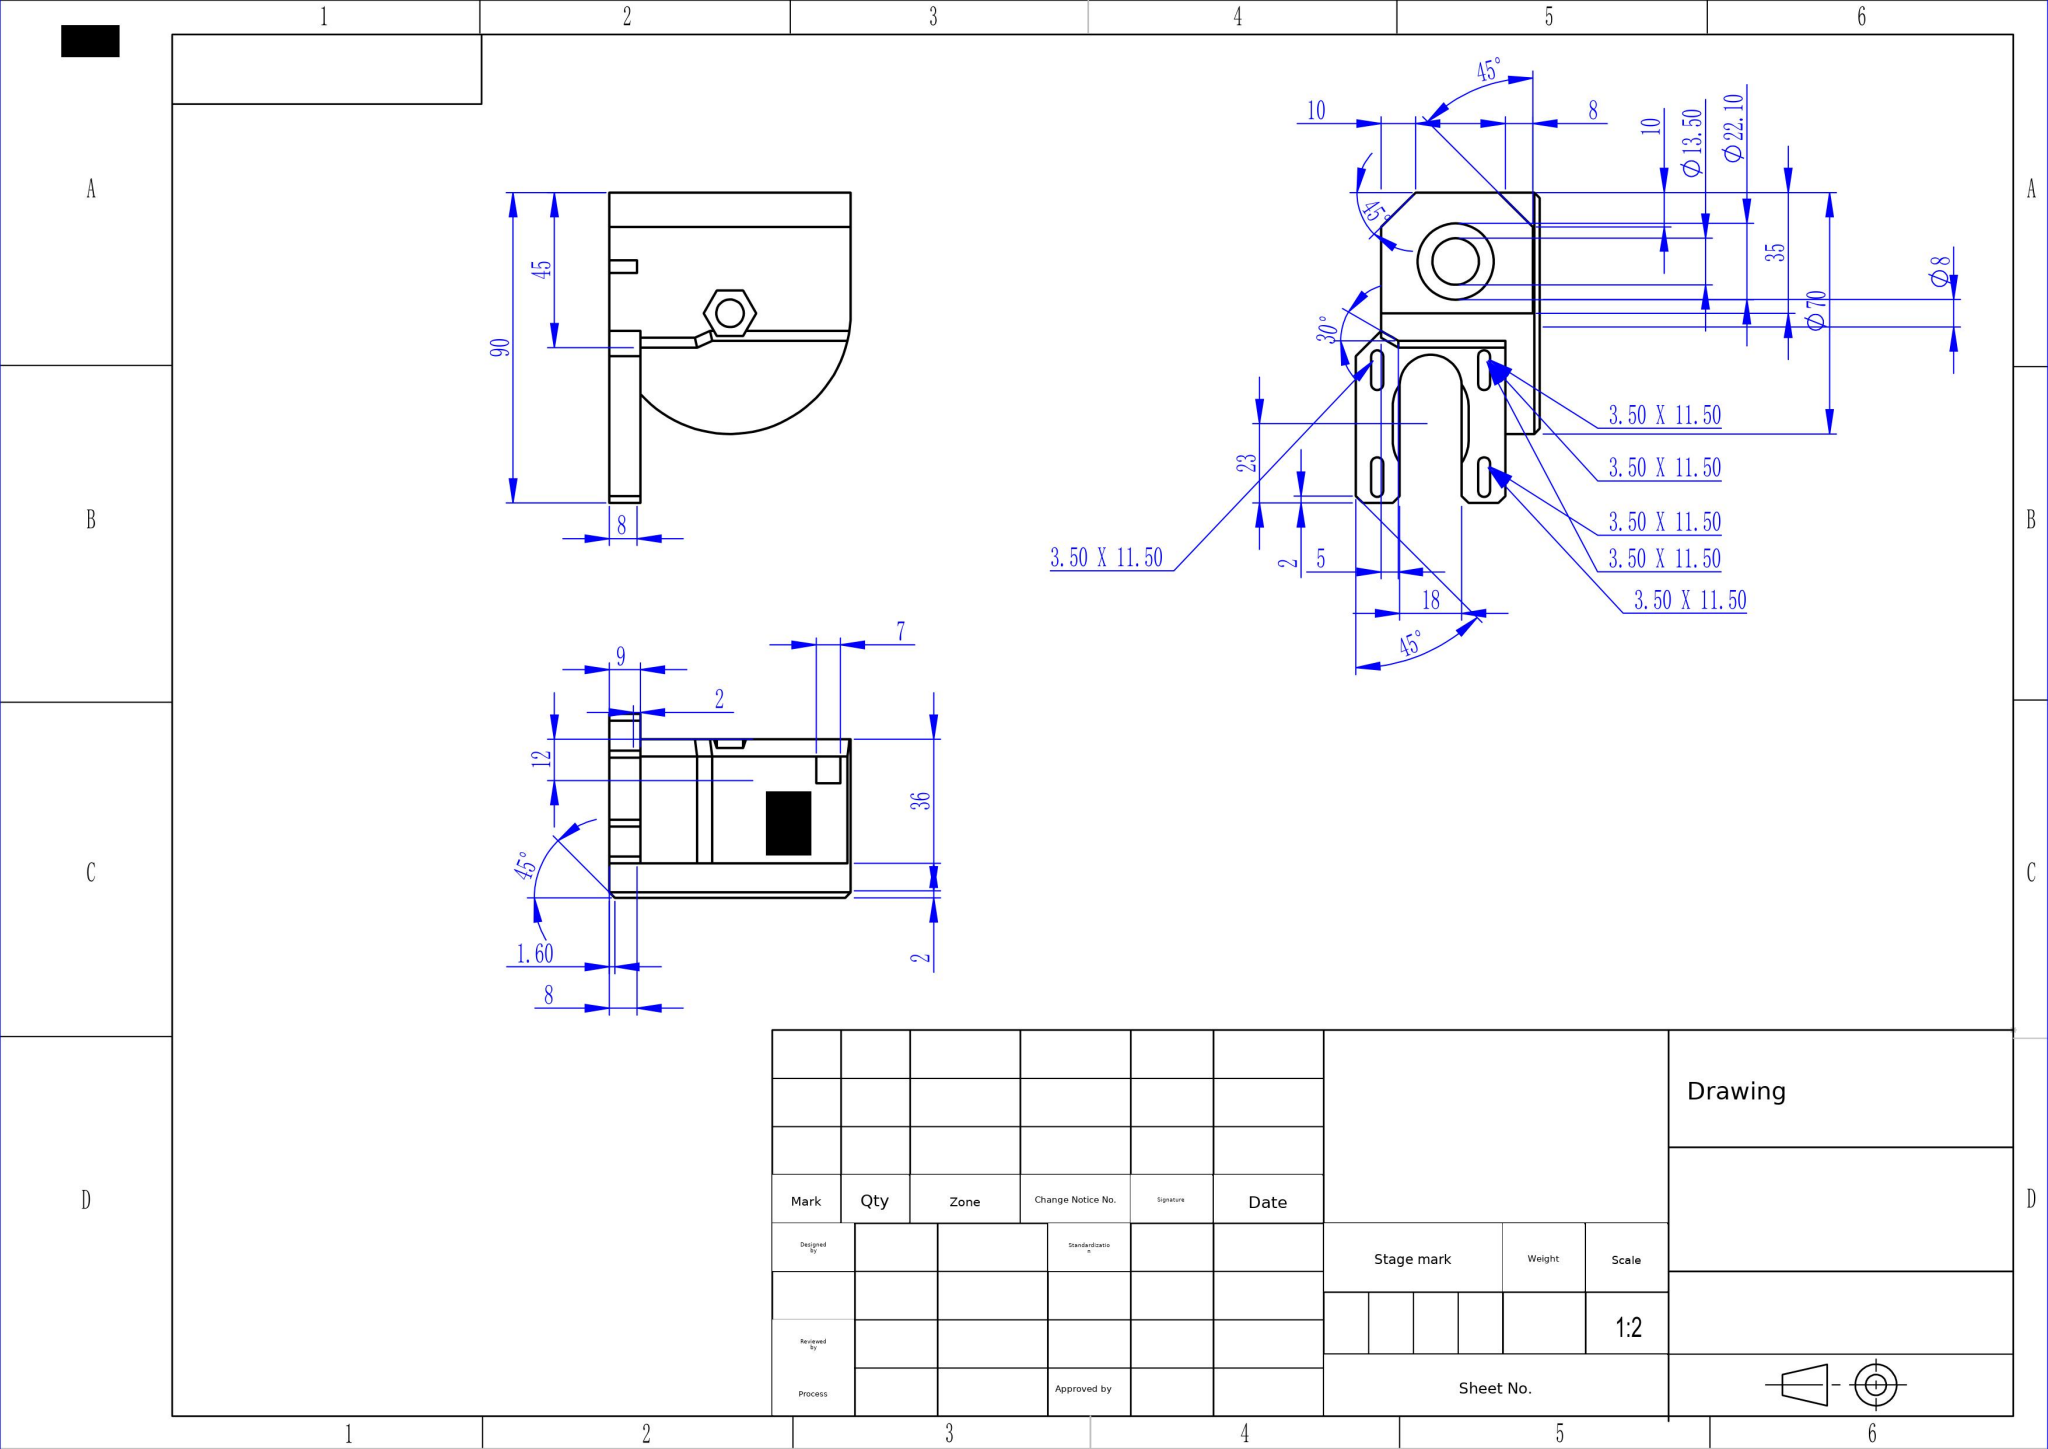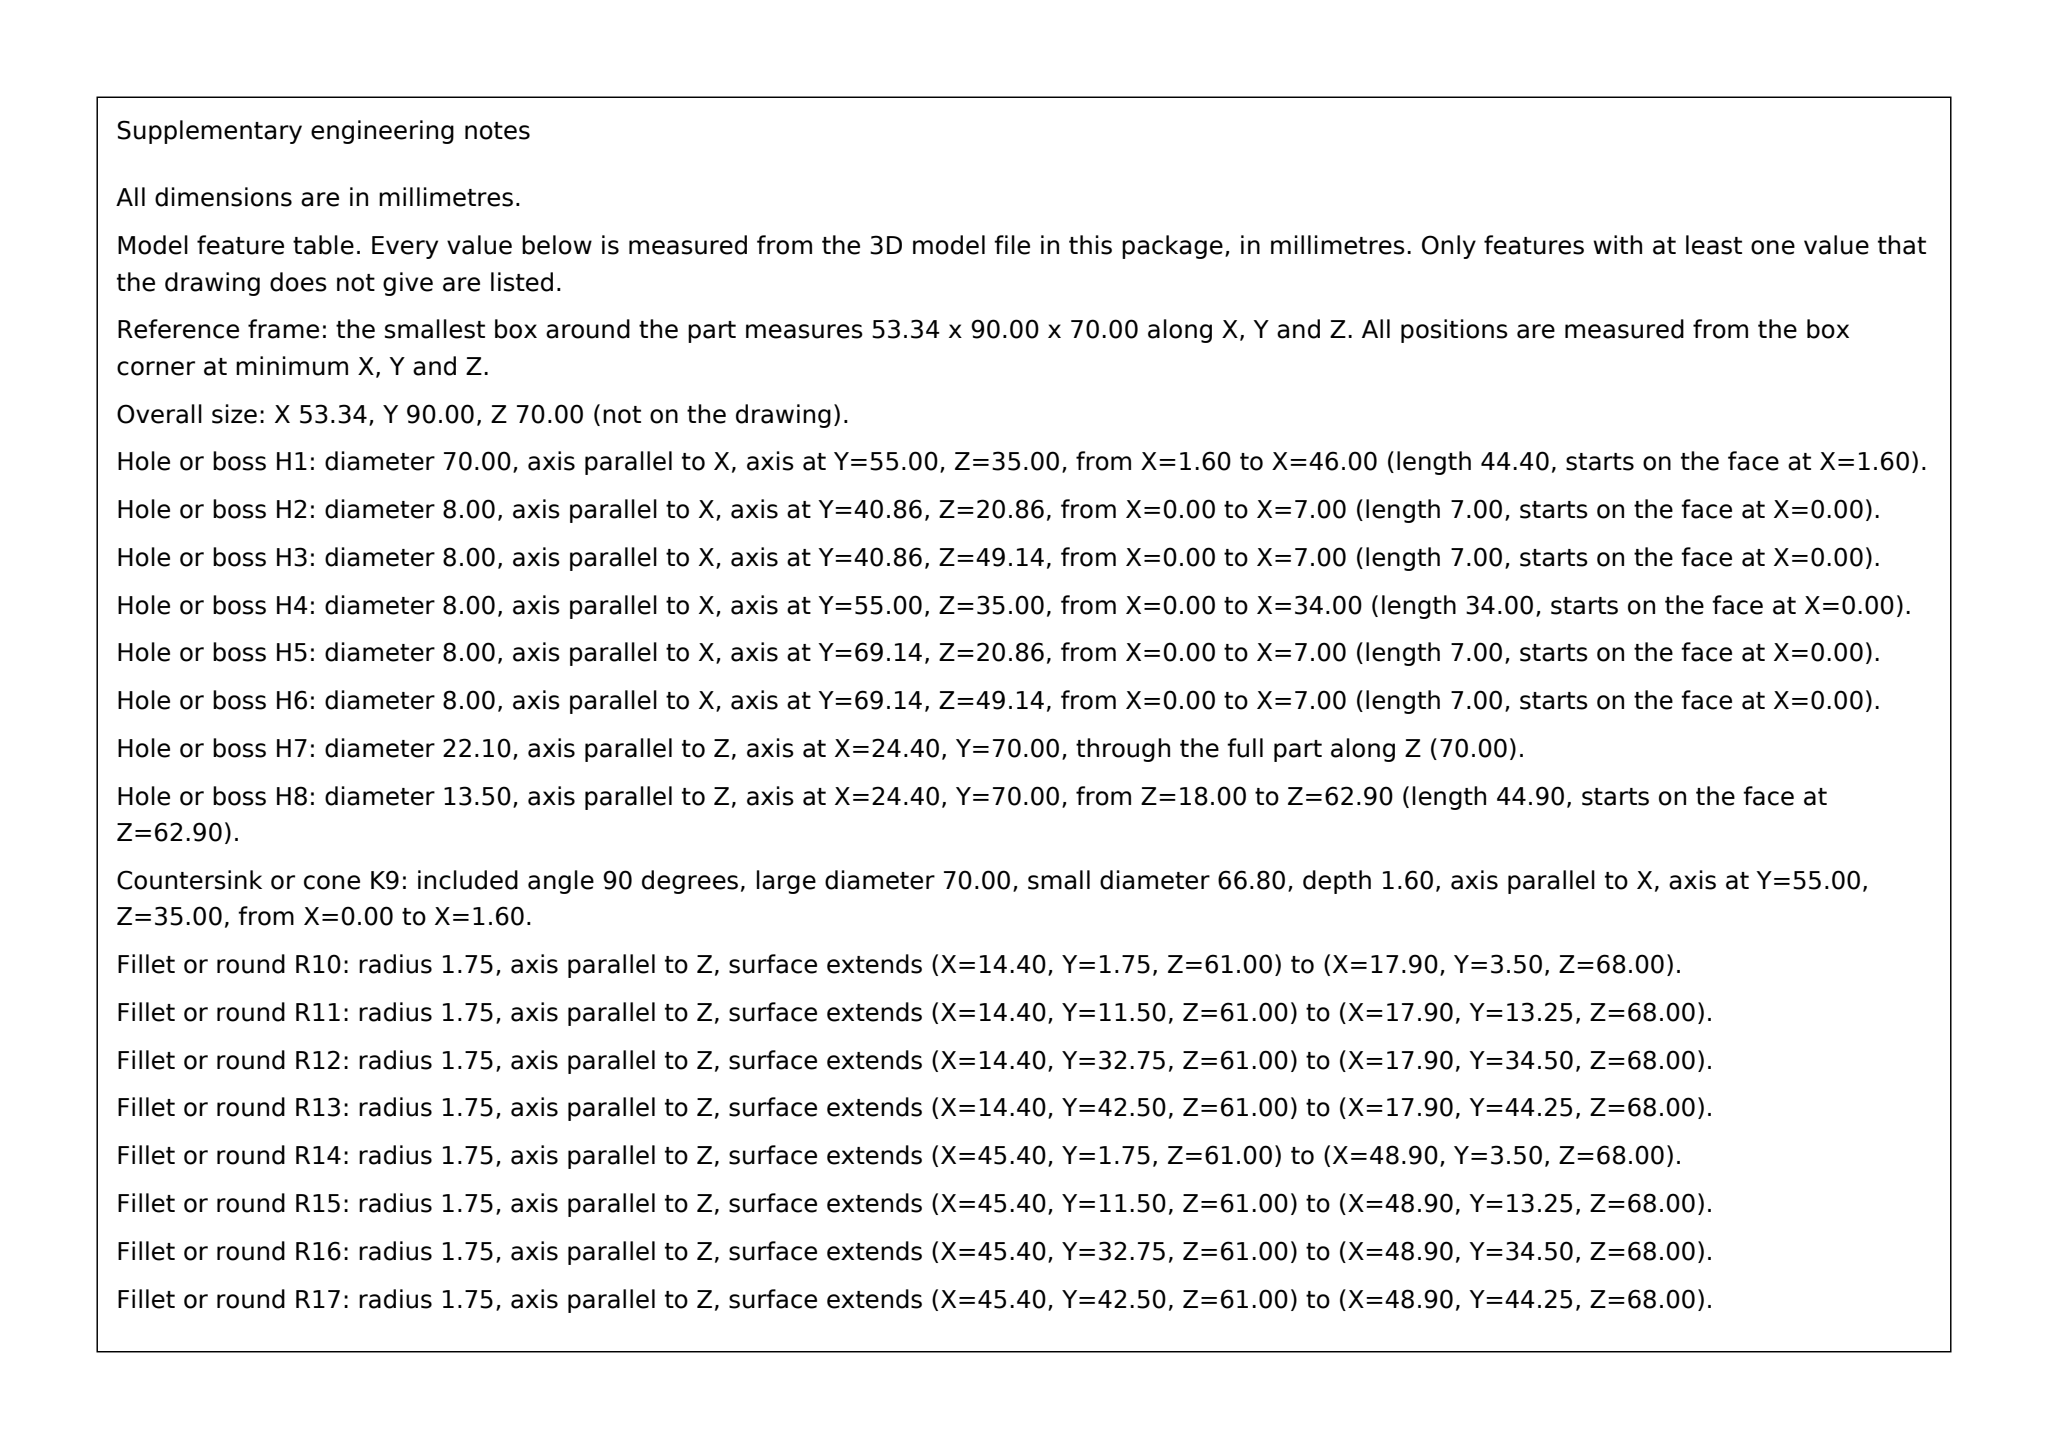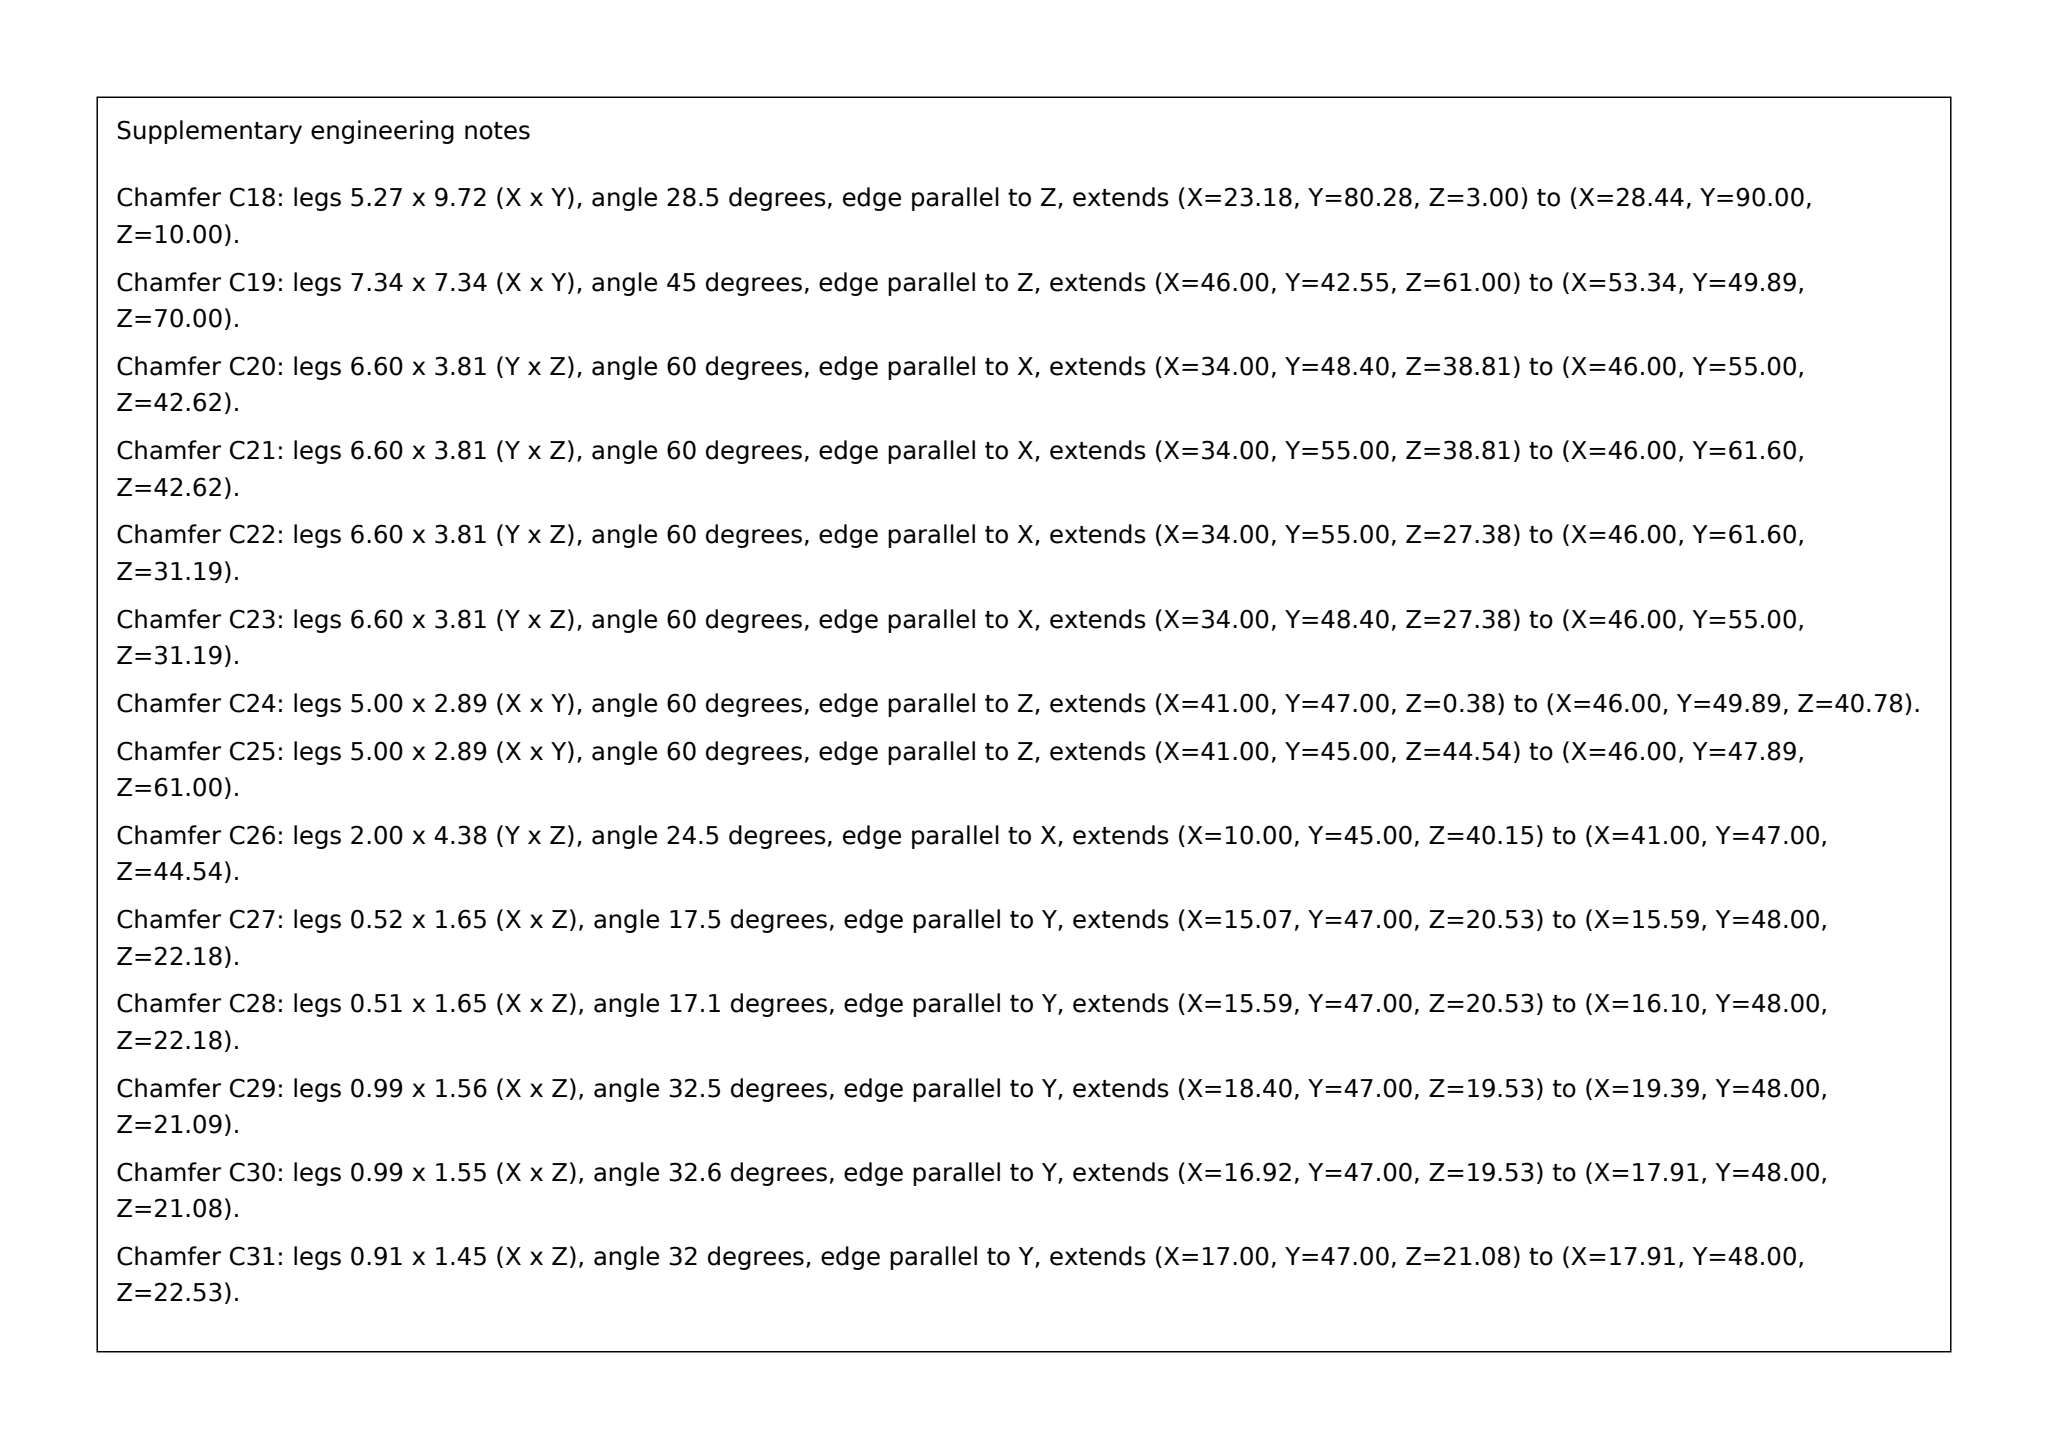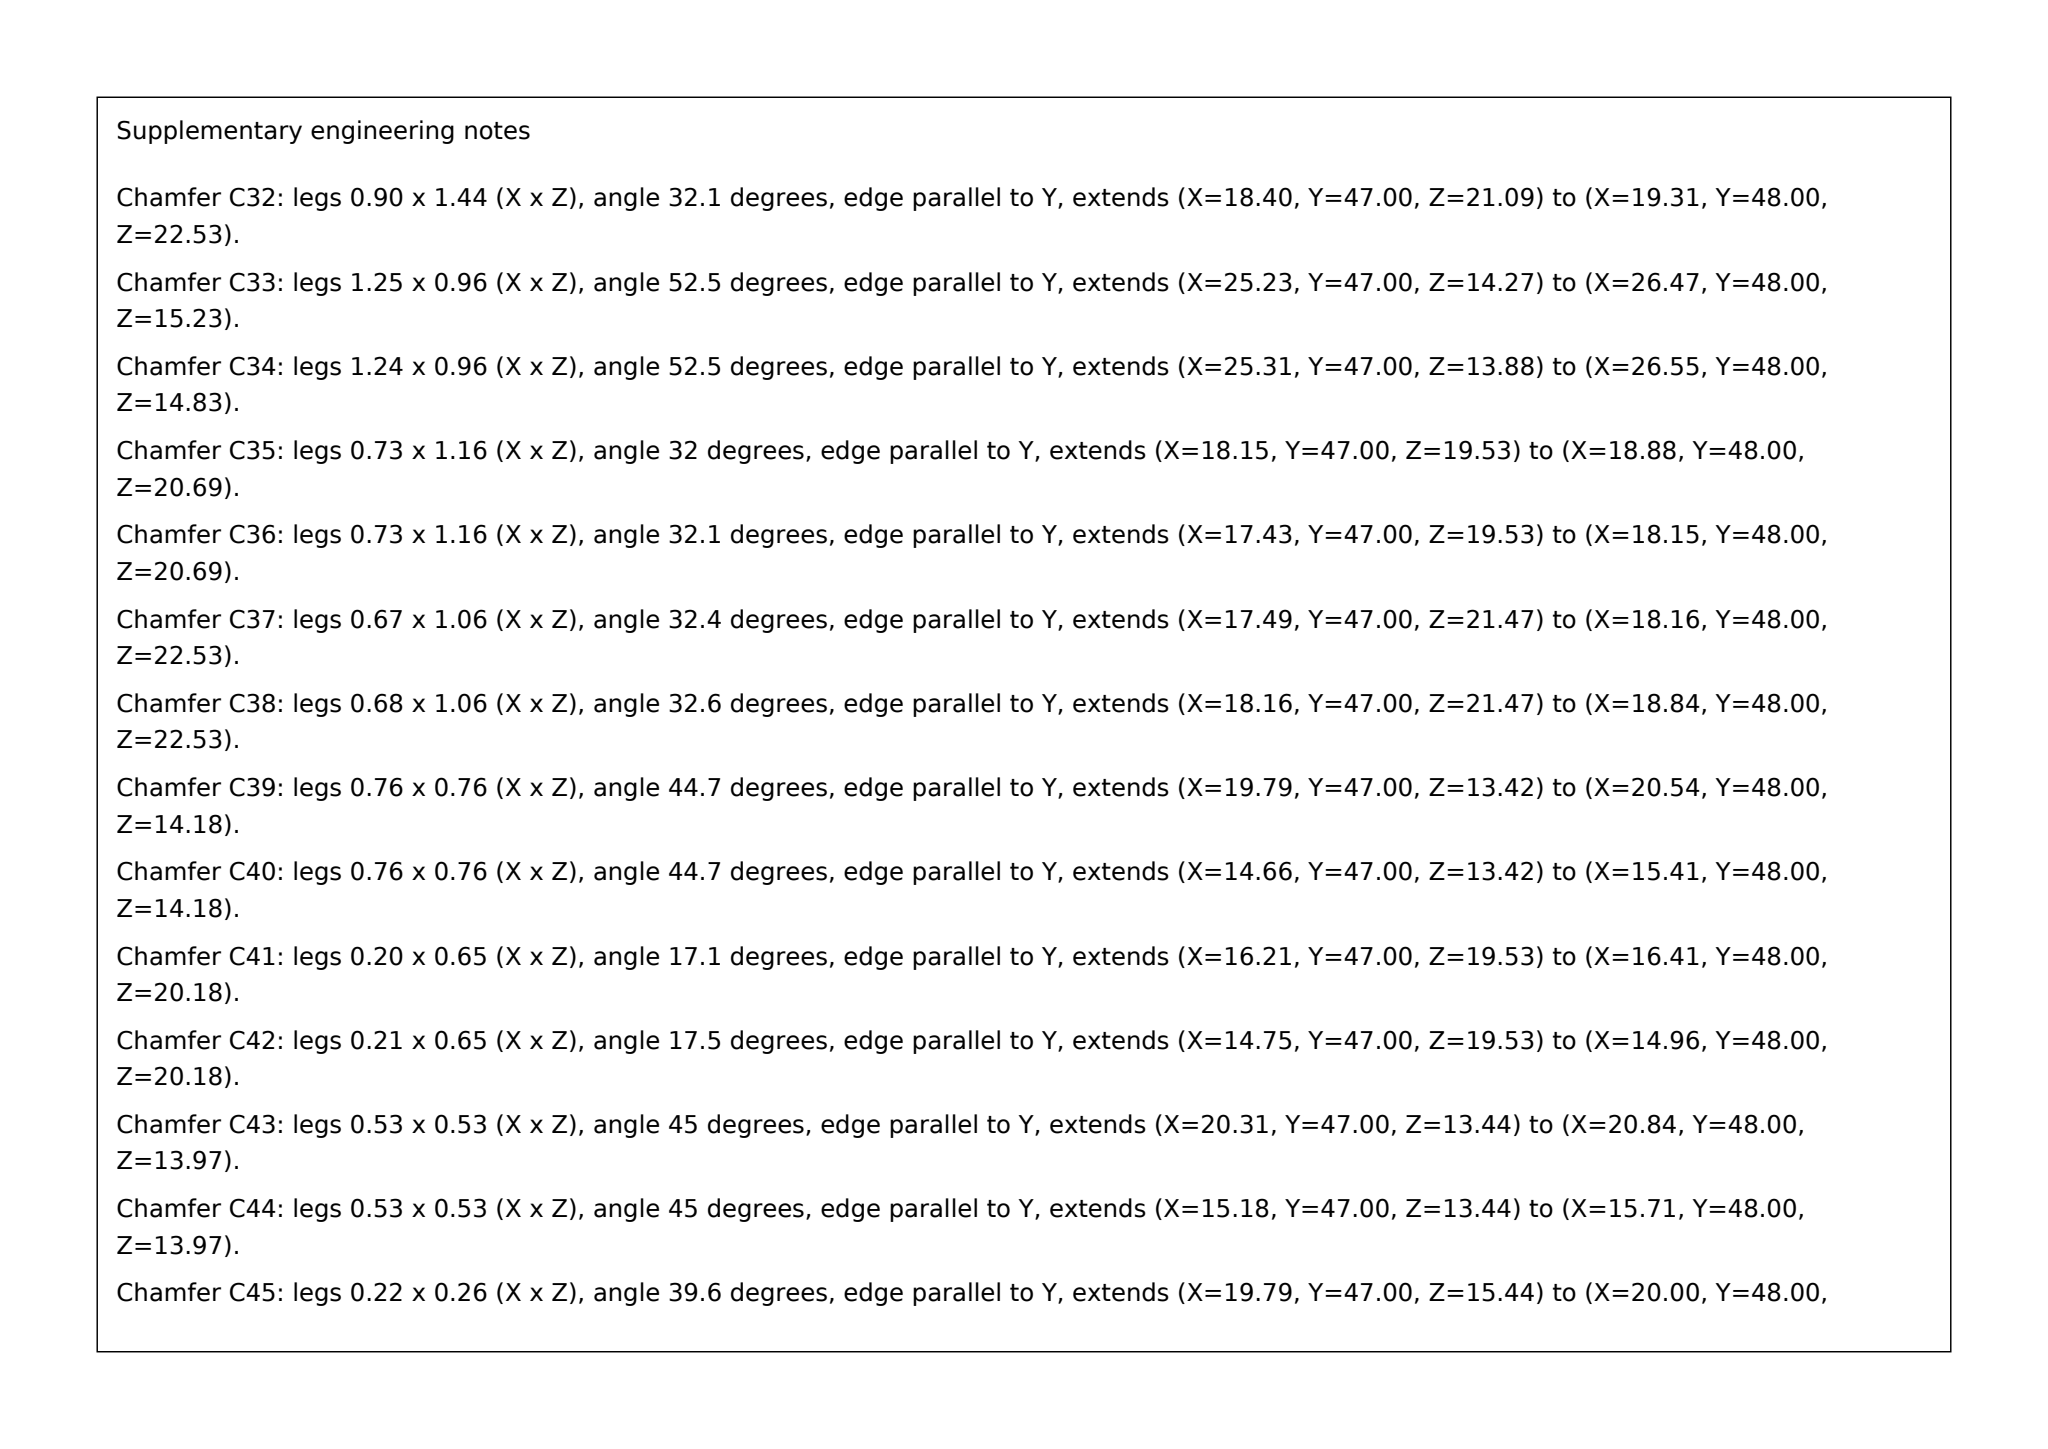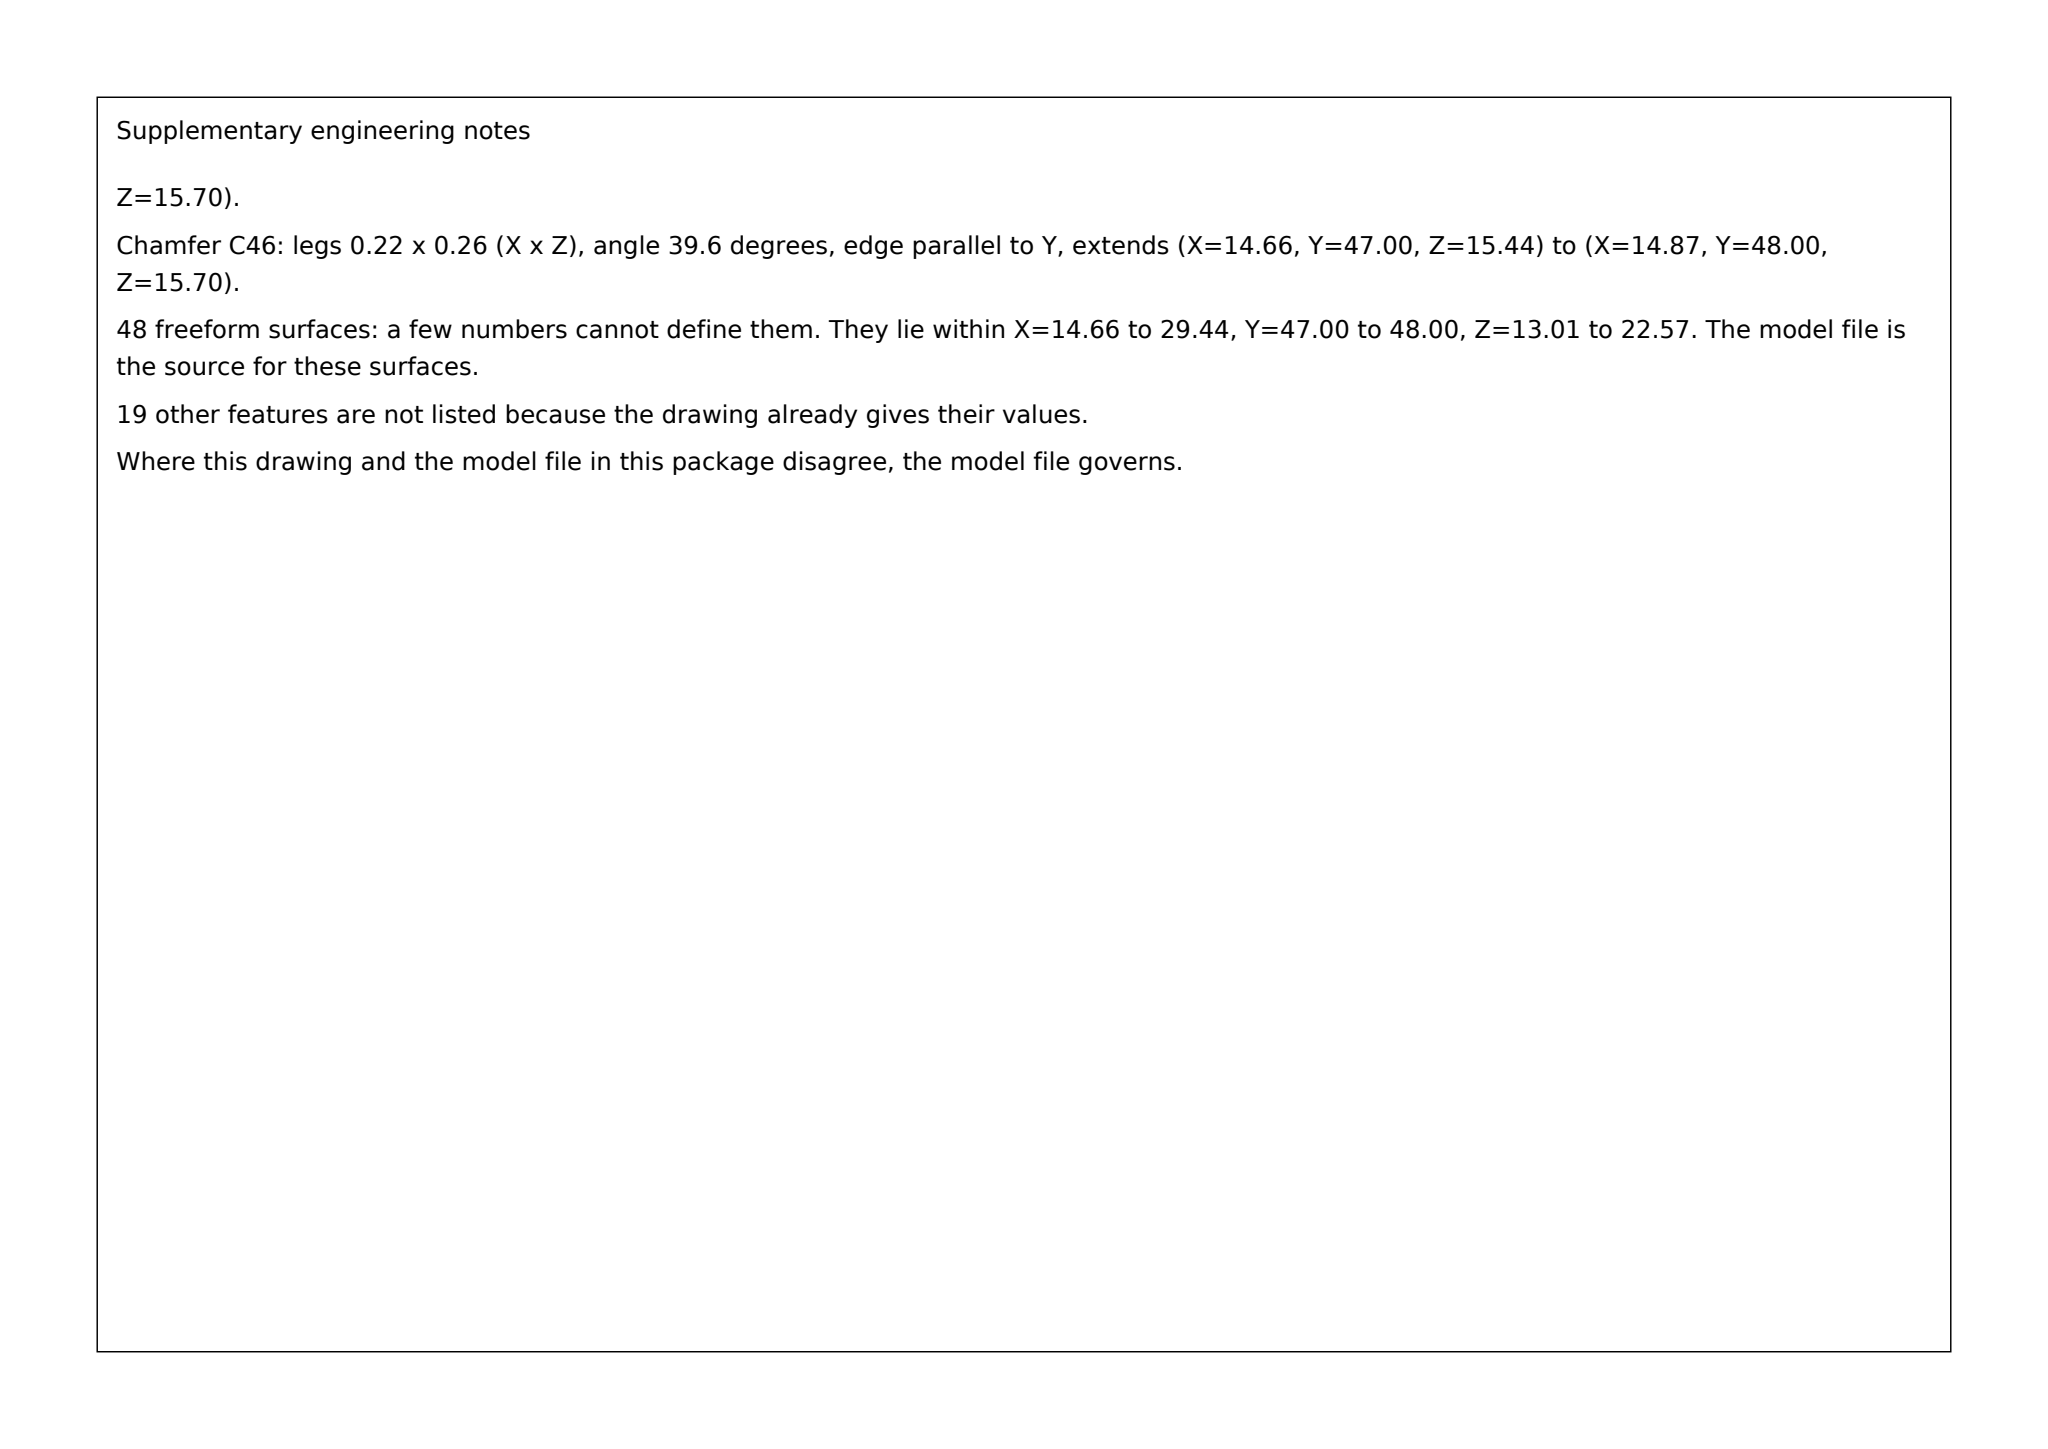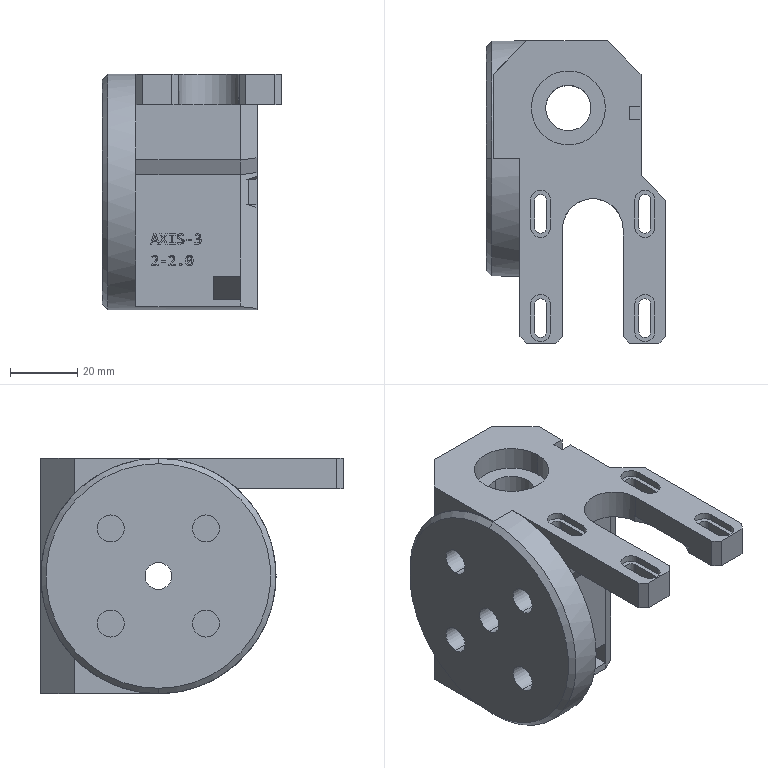Part | SolidWorks | mm | 1 solid | 245 faces | box 53.34 x 90 x 70 mm | volume 132479 mm3 | plane 156 | spline 48 | cylinder 39 | cone 2 | commonest cylinder face diameters 8 x10 3.5 x8 6 x8 22.1 x4 22 x4 70 x2 13.5 x2 18 x1